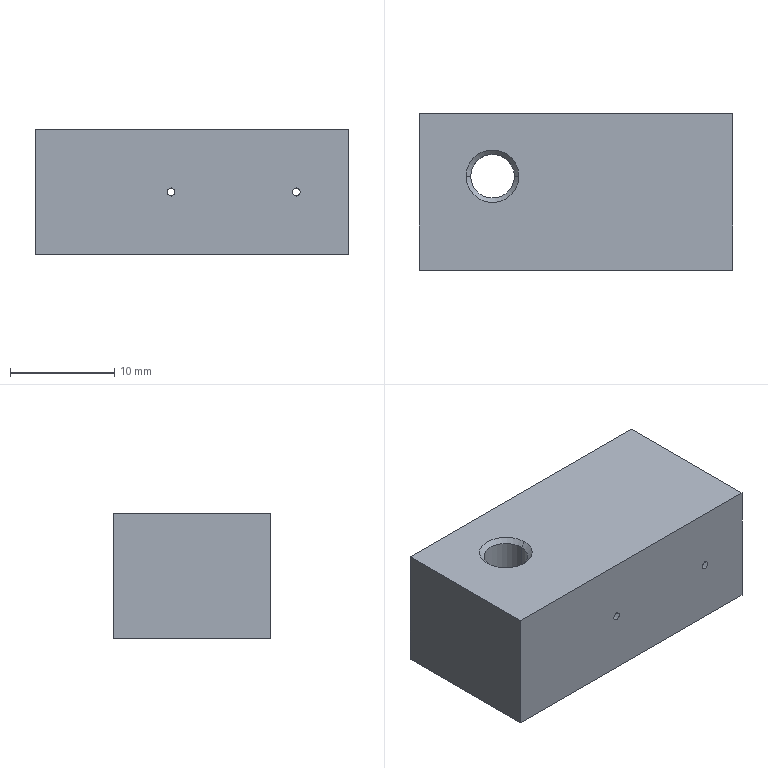CAM job | Mastercam | mm | 8 operations | part box 30 x 15 x 12
1. Facing | 20 - 63 平铣刀
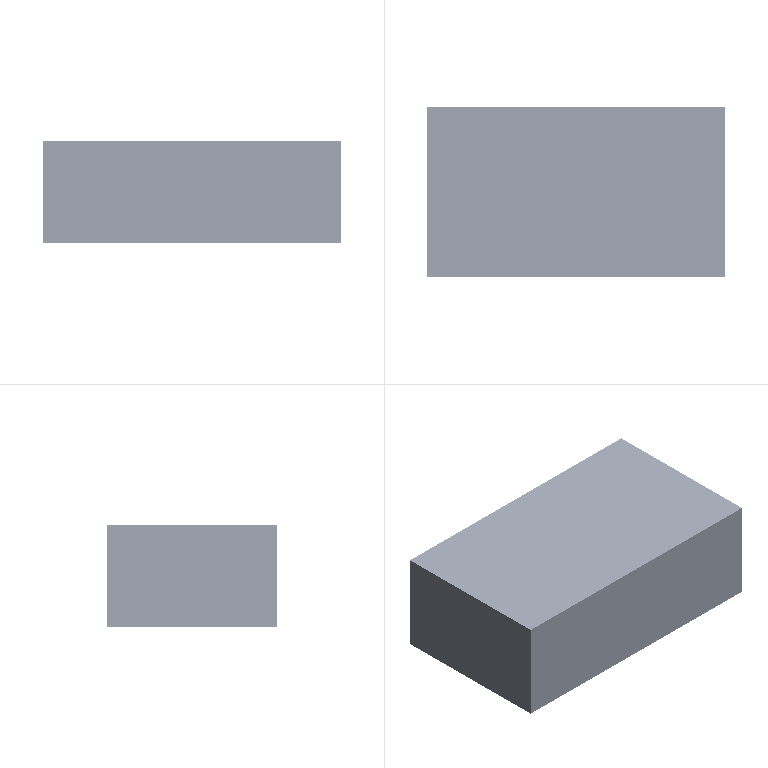2. Contour (Ramp) | 10 - 10 平铣刀
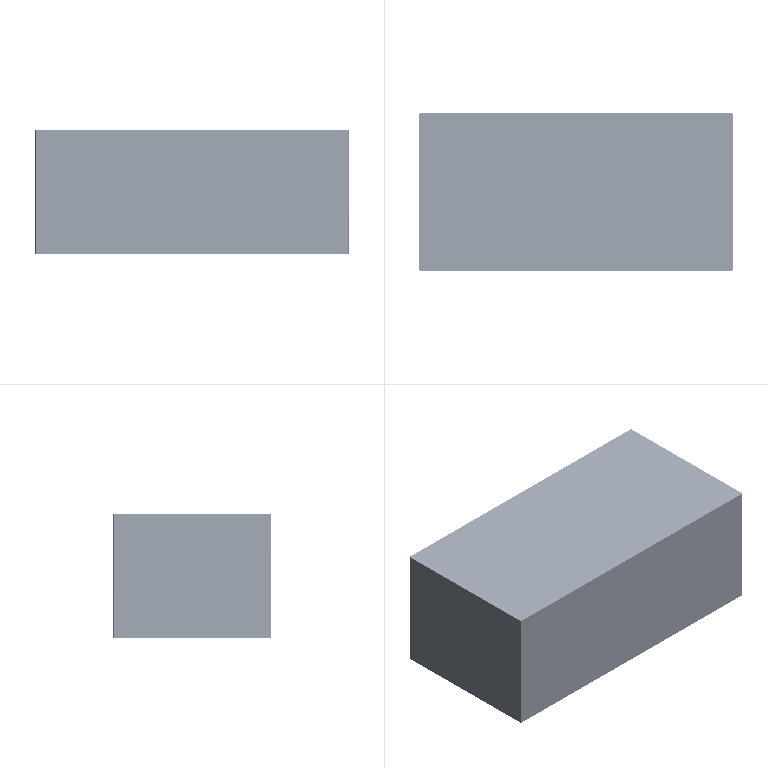3. Contour (2D) | 10 - 10 平铣刀
4. Contour (2D chamfer) | 7 - 4 倒角刀
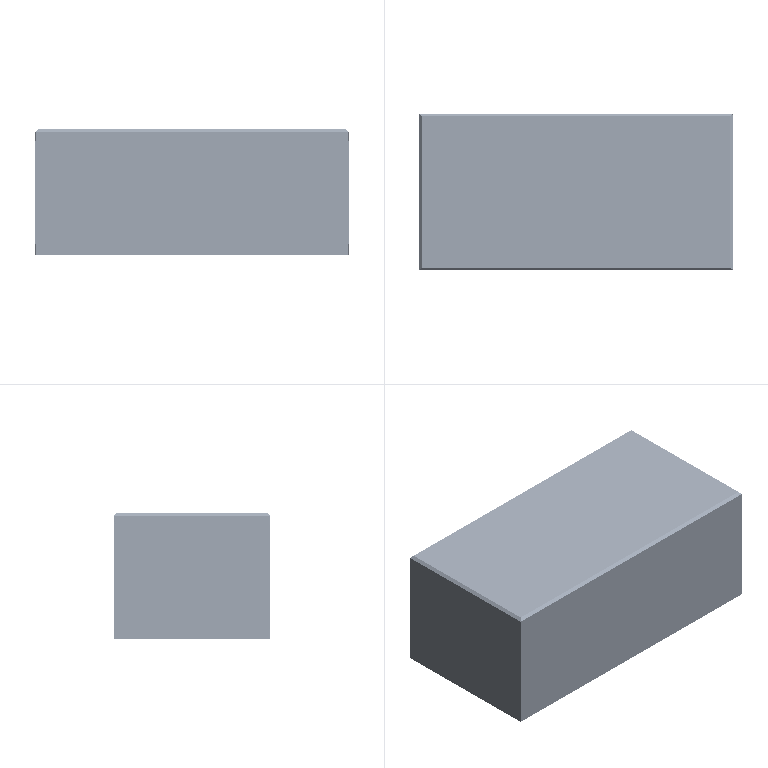5. Drill/Counterbore | 7 - 4 倒角刀
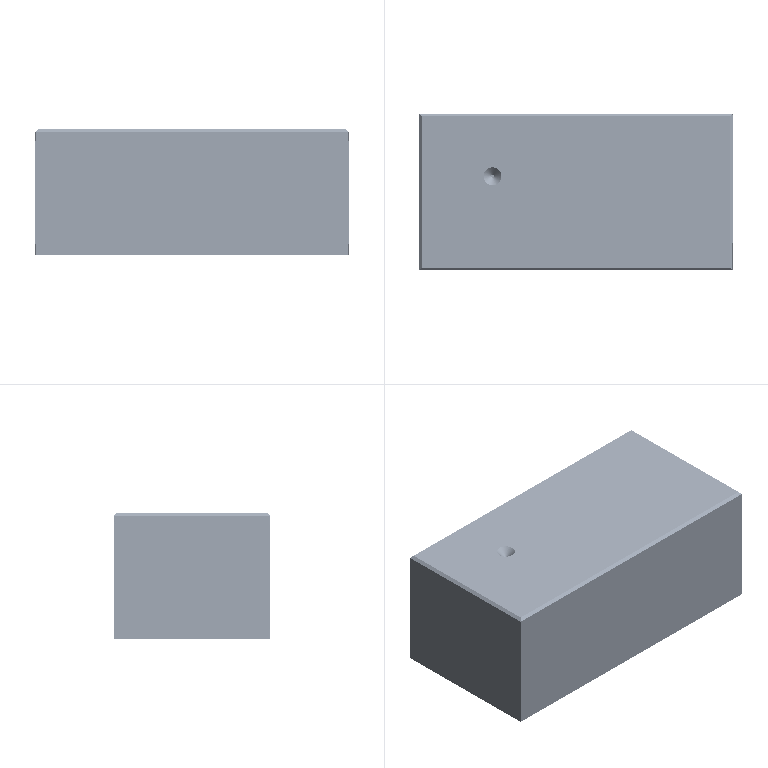6. Facing | 20 - 63 平铣刀
7. Contour (2D chamfer) | 7 - 4 倒角刀
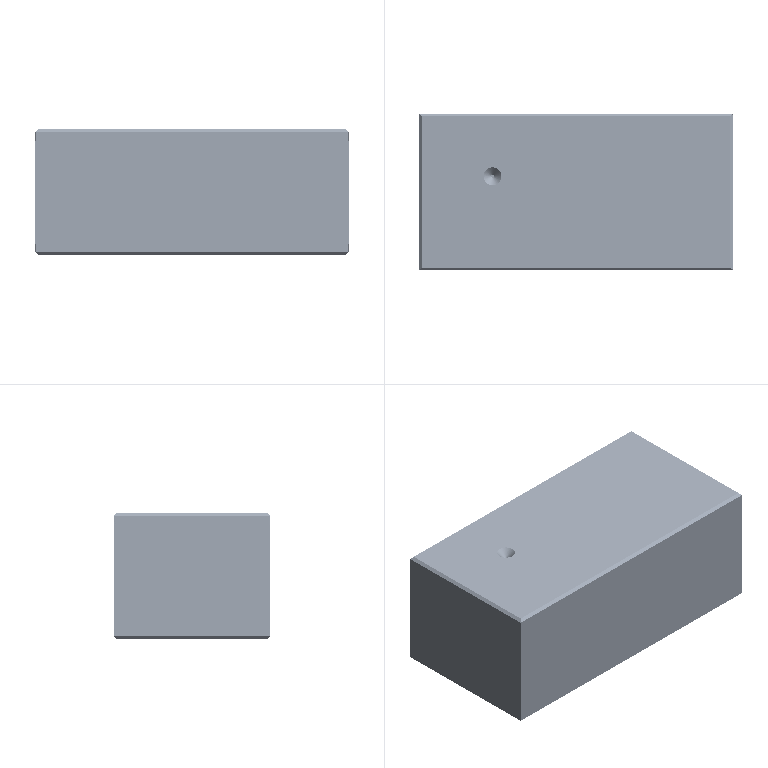8. Drill/Counterbore | 7 - 4 倒角刀